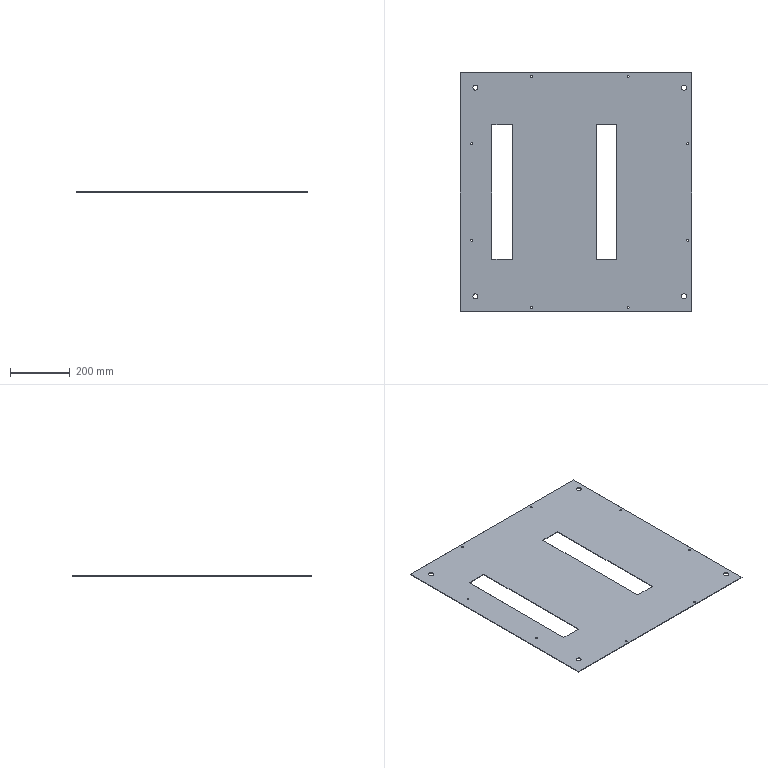Component | SolidWorks | TopPlate(Item8)-1 | 1 solid | 38 faces | volume 1111653 mm3 | cylinder 24 | plane 14 | commonest cylinder face diameters 6.5 x16 17 x8